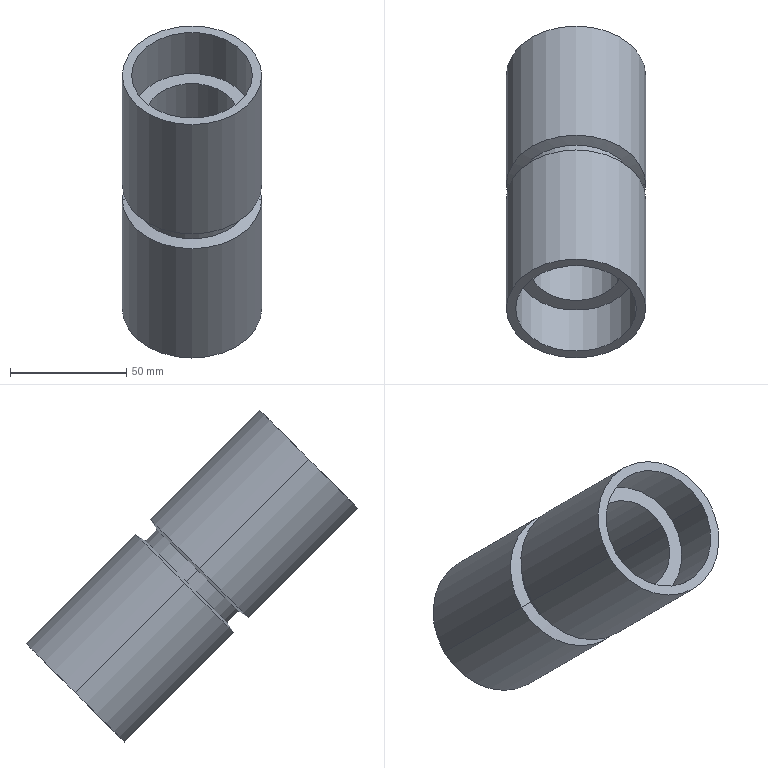Component | SolidWorks | PassiveRollerAssembly-1_StainlessSteelRoller-2 | 1 solid | 20 faces | box 60 x 142.84 x 142.84 mm | volume 167559 mm3 | cylinder 12 | cone 4 | plane 4 | commonest cylinder face diameters 52 x4 60 x4 40 x2 50 x2
build123d program:
from build123d import *


with BuildPart() as part:
    # Sketch1 → Revolve1 (revolve)
    with BuildSketch(Plane.XY, mode=Mode.PRIVATE) as revolve1_sk:
        Polygon((0, 26), (0, 30), (66.5, 30), (67.5, 25), (74.5, 25), (75.5, 30), (142, 30), (142, 26), (111, 26), (111, 20), (25, 20), (25, 26), align=None)
    revolve(revolve1_sk.sketch.rotate(Axis((-104.65, 0, 0), (1, 0, 0)), 90), axis=Axis((-104.65, 0, 0), (1, 0, 0)))


solid = part.part

# Placed as in the assembly
solid = solid.moved(Location((2216.026, 658.479, 246.908), (-45, -12.915, 90)))
STEP:
#1=COLOUR_RGB('',0.7922,0.8196,0.9333);
#2=FILL_AREA_STYLE_COLOUR('',#1);
#3=FILL_AREA_STYLE('',(#2));
#4=SURFACE_STYLE_FILL_AREA(#3);
#5=SURFACE_SIDE_STYLE('',(#4));
#6=SURFACE_STYLE_USAGE(.BOTH.,#5);
#7=PRESENTATION_STYLE_ASSIGNMENT((#6));
#8=CARTESIAN_POINT('',(86.458,29.014,6.631));
#9=VERTEX_POINT('',#8);
#10=CARTESIAN_POINT('',(88.033,29.014,6.631));
#11=VERTEX_POINT('',#10);
#12=CARTESIAN_POINT('',(87.245,29.014,6.631));
#13=DIRECTION('',(0.,-0.7071,0.7071));
#14=DIRECTION('',(1.,0.,0.));
#15=AXIS2_PLACEMENT_3D('',#12,#13,#14);
#16=CIRCLE('',#15,0.7874);
#17=EDGE_CURVE('',#9,#11,#16,.T.);
#18=ORIENTED_EDGE('',*,*,#17,.F.);
#19=CARTESIAN_POINT('',(86.458,26.62,9.025));
#20=VERTEX_POINT('',#19);
#21=CARTESIAN_POINT('',(86.458,23.011,12.634));
#22=DIRECTION('',(0.,-0.7071,0.7071));
#23=VECTOR('',#22,39.37);
#24=LINE('',#21,#23);
#25=EDGE_CURVE('',#9,#20,#24,.T.);
#26=ORIENTED_EDGE('',*,*,#25,.T.);
#27=CARTESIAN_POINT('',(88.033,26.62,9.025));
#28=VERTEX_POINT('',#27);
#29=CARTESIAN_POINT('',(87.245,26.62,9.025));
#30=DIRECTION('',(0.,-0.7071,0.7071));
#31=DIRECTION('',(1.,0.,0.));
#32=AXIS2_PLACEMENT_3D('',#29,#30,#31);
#33=CIRCLE('',#32,0.7874);
#34=EDGE_CURVE('',#20,#28,#33,.T.);
#35=ORIENTED_EDGE('',*,*,#34,.T.);
#36=CARTESIAN_POINT('',(88.033,23.011,12.634));
#37=DIRECTION('',(0.,-0.7071,0.7071));
#38=VECTOR('',#37,39.37);
#39=LINE('',#36,#38);
#40=EDGE_CURVE('',#11,#28,#39,.T.);
#41=ORIENTED_EDGE('',*,*,#40,.F.);
#42=EDGE_LOOP('',(#18,#26,#35,#41));
#43=FACE_OUTER_BOUND('',#42,.T.);
#44=CARTESIAN_POINT('',(87.245,23.011,12.634));
#45=DIRECTION('',(0.,-0.7071,0.7071));
#46=DIRECTION('',(1.,0.,0.));
#47=AXIS2_PLACEMENT_3D('',#44,#45,#46);
#48=CYLINDRICAL_SURFACE('',#47,0.7874);
#49=ADVANCED_FACE('',(#43),#48,.F.);
#50=CARTESIAN_POINT('',(86.222,29.877,5.768));
#51=VERTEX_POINT('',#50);
#52=CARTESIAN_POINT('',(88.269,29.877,5.768));
#53=VERTEX_POINT('',#52);
#54=CARTESIAN_POINT('',(87.245,29.877,5.768));
#55=DIRECTION('',(0.,-0.7071,0.7071));
#56=DIRECTION('',(1.,0.,0.));
#57=AXIS2_PLACEMENT_3D('',#54,#55,#56);
#58=CIRCLE('',#57,1.024);
#59=EDGE_CURVE('',#51,#53,#58,.T.);
#60=ORIENTED_EDGE('',*,*,#59,.F.);
#61=CARTESIAN_POINT('',(86.222,29.014,6.631));
#62=VERTEX_POINT('',#61);
#63=CARTESIAN_POINT('',(86.222,23.011,12.634));
#64=DIRECTION('',(0.,-0.7071,0.7071));
#65=VECTOR('',#64,39.37);
#66=LINE('',#63,#65);
#67=EDGE_CURVE('',#51,#62,#66,.T.);
#68=ORIENTED_EDGE('',*,*,#67,.T.);
#69=CARTESIAN_POINT('',(88.269,29.014,6.631));
#70=VERTEX_POINT('',#69);
#71=CARTESIAN_POINT('',(87.245,29.014,6.631));
#72=DIRECTION('',(0.,-0.7071,0.7071));
#73=DIRECTION('',(1.,0.,0.));
#74=AXIS2_PLACEMENT_3D('',#71,#72,#73);
#75=CIRCLE('',#74,1.024);
#76=EDGE_CURVE('',#62,#70,#75,.T.);
#77=ORIENTED_EDGE('',*,*,#76,.T.);
#78=CARTESIAN_POINT('',(88.269,23.011,12.634));
#79=DIRECTION('',(0.,-0.7071,0.7071));
#80=VECTOR('',#79,39.37);
#81=LINE('',#78,#80);
#82=EDGE_CURVE('',#53,#70,#81,.T.);
#83=ORIENTED_EDGE('',*,*,#82,.F.);
#84=EDGE_LOOP('',(#60,#68,#77,#83));
#85=FACE_OUTER_BOUND('',#84,.T.);
#86=CARTESIAN_POINT('',(87.245,23.011,12.634));
#87=DIRECTION('',(0.,-0.7071,0.7071));
#88=DIRECTION('',(1.,0.,0.));
#89=AXIS2_PLACEMENT_3D('',#86,#87,#88);
#90=CYLINDRICAL_SURFACE('',#89,1.024);
#91=ADVANCED_FACE('',(#85),#90,.F.);
#92=CARTESIAN_POINT('',(88.426,29.877,5.768));
#93=VERTEX_POINT('',#92);
#94=CARTESIAN_POINT('',(86.064,29.877,5.768));
#95=VERTEX_POINT('',#94);
#96=CARTESIAN_POINT('',(87.245,29.877,5.768));
#97=DIRECTION('',(0.,-0.7071,0.7071));
#98=DIRECTION('',(1.,0.,0.));
#99=AXIS2_PLACEMENT_3D('',#96,#97,#98);
#100=CIRCLE('',#99,1.181);
#101=EDGE_CURVE('',#93,#95,#100,.T.);
#102=ORIENTED_EDGE('',*,*,#101,.T.);
#103=CARTESIAN_POINT('',(86.064,28.026,7.619));
#104=VERTEX_POINT('',#103);
#105=CARTESIAN_POINT('',(86.064,23.011,12.634));
#106=DIRECTION('',(0.,-0.7071,0.7071));
#107=VECTOR('',#106,39.37);
#108=LINE('',#105,#107);
#109=EDGE_CURVE('',#95,#104,#108,.T.);
#110=ORIENTED_EDGE('',*,*,#109,.T.);
#111=CARTESIAN_POINT('',(88.426,28.026,7.619));
#112=VERTEX_POINT('',#111);
#113=CARTESIAN_POINT('',(87.245,28.026,7.619));
#114=DIRECTION('',(0.,-0.7071,0.7071));
#115=DIRECTION('',(1.,0.,0.));
#116=AXIS2_PLACEMENT_3D('',#113,#114,#115);
#117=CIRCLE('',#116,1.181);
#118=EDGE_CURVE('',#112,#104,#117,.T.);
#119=ORIENTED_EDGE('',*,*,#118,.F.);
#120=CARTESIAN_POINT('',(88.426,23.011,12.634));
#121=DIRECTION('',(0.,-0.7071,0.7071));
#122=VECTOR('',#121,39.37);
#123=LINE('',#120,#122);
#124=EDGE_CURVE('',#93,#112,#123,.T.);
#125=ORIENTED_EDGE('',*,*,#124,.F.);
#126=EDGE_LOOP('',(#102,#110,#119,#125));
#127=FACE_OUTER_BOUND('',#126,.T.);
#128=CARTESIAN_POINT('',(87.245,23.011,12.634));
#129=DIRECTION('',(0.,-0.7071,0.7071));
#130=DIRECTION('',(1.,0.,0.));
#131=AXIS2_PLACEMENT_3D('',#128,#129,#130);
#132=CYLINDRICAL_SURFACE('',#131,1.181);
#133=ADVANCED_FACE('',(#127),#132,.T.);
#134=CARTESIAN_POINT('',(88.229,27.998,7.647));
#135=VERTEX_POINT('',#134);
#136=CARTESIAN_POINT('',(86.261,27.998,7.647));
#137=VERTEX_POINT('',#136);
#138=CARTESIAN_POINT('',(87.245,27.998,7.647));
#139=DIRECTION('',(0.,-0.7071,0.7071));
#140=DIRECTION('',(1.,0.,0.));
#141=AXIS2_PLACEMENT_3D('',#138,#139,#140);
#142=CIRCLE('',#141,0.9843);
#143=EDGE_CURVE('',#135,#137,#142,.T.);
#144=ORIENTED_EDGE('',*,*,#143,.F.);
#145=CARTESIAN_POINT('',(88.426,28.026,7.619));
#146=DIRECTION('',(0.9806,0.1387,-0.1387));
#147=VECTOR('',#146,39.37);
#148=LINE('',#145,#147);
#149=EDGE_CURVE('',#135,#112,#148,.T.);
#150=ORIENTED_EDGE('',*,*,#149,.T.);
#151=ORIENTED_EDGE('',*,*,#118,.T.);
#152=CARTESIAN_POINT('',(86.064,28.026,7.619));
#153=DIRECTION('',(-0.9806,0.1387,-0.1387));
#154=VECTOR('',#153,39.37);
#155=LINE('',#152,#154);
#156=EDGE_CURVE('',#137,#104,#155,.T.);
#157=ORIENTED_EDGE('',*,*,#156,.F.);
#158=EDGE_LOOP('',(#144,#150,#151,#157));
#159=FACE_OUTER_BOUND('',#158,.T.);
#160=CARTESIAN_POINT('',(87.245,28.026,7.619));
#161=DIRECTION('',(-0.,0.7071,-0.7071));
#162=DIRECTION('',(-1.,0.,0.));
#163=AXIS2_PLACEMENT_3D('',#160,#161,#162);
#164=CONICAL_SURFACE('',#163,1.181,1.373);
#165=ADVANCED_FACE('',(#159),#164,.T.);
#166=ORIENTED_EDGE('',*,*,#143,.T.);
#167=CARTESIAN_POINT('',(86.261,27.803,7.842));
#168=VERTEX_POINT('',#167);
#169=CARTESIAN_POINT('',(86.261,23.011,12.634));
#170=DIRECTION('',(0.,-0.7071,0.7071));
#171=VECTOR('',#170,39.37);
#172=LINE('',#169,#171);
#173=EDGE_CURVE('',#137,#168,#172,.T.);
#174=ORIENTED_EDGE('',*,*,#173,.T.);
#175=CARTESIAN_POINT('',(88.229,27.803,7.842));
#176=VERTEX_POINT('',#175);
#177=CARTESIAN_POINT('',(87.245,27.803,7.842));
#178=DIRECTION('',(0.,-0.7071,0.7071));
#179=DIRECTION('',(1.,0.,0.));
#180=AXIS2_PLACEMENT_3D('',#177,#178,#179);
#181=CIRCLE('',#180,0.9843);
#182=EDGE_CURVE('',#176,#168,#181,.T.);
#183=ORIENTED_EDGE('',*,*,#182,.F.);
#184=CARTESIAN_POINT('',(88.229,23.011,12.634));
#185=DIRECTION('',(0.,-0.7071,0.7071));
#186=VECTOR('',#185,39.37);
#187=LINE('',#184,#186);
#188=EDGE_CURVE('',#135,#176,#187,.T.);
#189=ORIENTED_EDGE('',*,*,#188,.F.);
#190=EDGE_LOOP('',(#166,#174,#183,#189));
#191=FACE_OUTER_BOUND('',#190,.T.);
#192=CARTESIAN_POINT('',(87.245,23.011,12.634));
#193=DIRECTION('',(0.,-0.7071,0.7071));
#194=DIRECTION('',(1.,0.,0.));
#195=AXIS2_PLACEMENT_3D('',#192,#193,#194);
#196=CYLINDRICAL_SURFACE('',#195,0.9843);
#197=ADVANCED_FACE('',(#191),#196,.T.);
#198=ORIENTED_EDGE('',*,*,#182,.T.);
#199=CARTESIAN_POINT('',(86.064,27.776,7.87));
#200=VERTEX_POINT('',#199);
#201=CARTESIAN_POINT('',(86.261,27.803,7.842));
#202=DIRECTION('',(-0.9806,-0.1387,0.1387));
#203=VECTOR('',#202,39.37);
#204=LINE('',#201,#203);
#205=EDGE_CURVE('',#168,#200,#204,.T.);
#206=ORIENTED_EDGE('',*,*,#205,.T.);
#207=CARTESIAN_POINT('',(88.426,27.776,7.87));
#208=VERTEX_POINT('',#207);
#209=CARTESIAN_POINT('',(87.245,27.776,7.87));
#210=DIRECTION('',(0.,-0.7071,0.7071));
#211=DIRECTION('',(1.,0.,0.));
#212=AXIS2_PLACEMENT_3D('',#209,#210,#211);
#213=CIRCLE('',#212,1.181);
#214=EDGE_CURVE('',#208,#200,#213,.T.);
#215=ORIENTED_EDGE('',*,*,#214,.F.);
#216=CARTESIAN_POINT('',(88.229,27.803,7.842));
#217=DIRECTION('',(0.9806,-0.1387,0.1387));
#218=VECTOR('',#217,39.37);
#219=LINE('',#216,#218);
#220=EDGE_CURVE('',#176,#208,#219,.T.);
#221=ORIENTED_EDGE('',*,*,#220,.F.);
#222=EDGE_LOOP('',(#198,#206,#215,#221));
#223=FACE_OUTER_BOUND('',#222,.T.);
#224=CARTESIAN_POINT('',(87.245,27.803,7.842));
#225=DIRECTION('',(0.,-0.7071,0.7071));
#226=DIRECTION('',(1.,0.,0.));
#227=AXIS2_PLACEMENT_3D('',#224,#225,#226);
#228=CONICAL_SURFACE('',#227,0.9843,1.373);
#229=ADVANCED_FACE('',(#223),#228,.T.);
#230=ORIENTED_EDGE('',*,*,#214,.T.);
#231=CARTESIAN_POINT('',(86.064,25.924,9.721));
#232=VERTEX_POINT('',#231);
#233=CARTESIAN_POINT('',(86.064,23.011,12.634));
#234=DIRECTION('',(0.,-0.7071,0.7071));
#235=VECTOR('',#234,39.37);
#236=LINE('',#233,#235);
#237=EDGE_CURVE('',#200,#232,#236,.T.);
#238=ORIENTED_EDGE('',*,*,#237,.T.);
#239=CARTESIAN_POINT('',(88.426,25.924,9.721));
#240=VERTEX_POINT('',#239);
#241=CARTESIAN_POINT('',(87.245,25.924,9.721));
#242=DIRECTION('',(0.,-0.7071,0.7071));
#243=DIRECTION('',(1.,0.,0.));
#244=AXIS2_PLACEMENT_3D('',#241,#242,#243);
#245=CIRCLE('',#244,1.181);
#246=EDGE_CURVE('',#240,#232,#245,.T.);
#247=ORIENTED_EDGE('',*,*,#246,.F.);
#248=CARTESIAN_POINT('',(88.426,23.011,12.634));
#249=DIRECTION('',(0.,-0.7071,0.7071));
#250=VECTOR('',#249,39.37);
#251=LINE('',#248,#250);
#252=EDGE_CURVE('',#208,#240,#251,.T.);
#253=ORIENTED_EDGE('',*,*,#252,.F.);
#254=EDGE_LOOP('',(#230,#238,#247,#253));
#255=FACE_OUTER_BOUND('',#254,.T.);
#256=CARTESIAN_POINT('',(87.245,23.011,12.634));
#257=DIRECTION('',(0.,-0.7071,0.7071));
#258=DIRECTION('',(1.,0.,0.));
#259=AXIS2_PLACEMENT_3D('',#256,#257,#258);
#260=CYLINDRICAL_SURFACE('',#259,1.181);
#261=ADVANCED_FACE('',(#255),#260,.T.);
#262=CARTESIAN_POINT('',(86.222,26.62,9.025));
#263=VERTEX_POINT('',#262);
#264=CARTESIAN_POINT('',(88.269,26.62,9.025));
#265=VERTEX_POINT('',#264);
#266=CARTESIAN_POINT('',(87.245,26.62,9.025));
#267=DIRECTION('',(0.,-0.7071,0.7071));
#268=DIRECTION('',(1.,0.,0.));
#269=AXIS2_PLACEMENT_3D('',#266,#267,#268);
#270=CIRCLE('',#269,1.024);
#271=EDGE_CURVE('',#263,#265,#270,.T.);
#272=ORIENTED_EDGE('',*,*,#271,.F.);
#273=CARTESIAN_POINT('',(86.222,25.924,9.721));
#274=VERTEX_POINT('',#273);
#275=CARTESIAN_POINT('',(86.222,23.011,12.634));
#276=DIRECTION('',(0.,-0.7071,0.7071));
#277=VECTOR('',#276,39.37);
#278=LINE('',#275,#277);
#279=EDGE_CURVE('',#263,#274,#278,.T.);
#280=ORIENTED_EDGE('',*,*,#279,.T.);
#281=CARTESIAN_POINT('',(88.269,25.924,9.721));
#282=VERTEX_POINT('',#281);
#283=CARTESIAN_POINT('',(87.245,25.924,9.721));
#284=DIRECTION('',(0.,-0.7071,0.7071));
#285=DIRECTION('',(1.,0.,0.));
#286=AXIS2_PLACEMENT_3D('',#283,#284,#285);
#287=CIRCLE('',#286,1.024);
#288=EDGE_CURVE('',#274,#282,#287,.T.);
#289=ORIENTED_EDGE('',*,*,#288,.T.);
#290=CARTESIAN_POINT('',(88.269,23.011,12.634));
#291=DIRECTION('',(0.,-0.7071,0.7071));
#292=VECTOR('',#291,39.37);
#293=LINE('',#290,#292);
#294=EDGE_CURVE('',#265,#282,#293,.T.);
#295=ORIENTED_EDGE('',*,*,#294,.F.);
#296=EDGE_LOOP('',(#272,#280,#289,#295));
#297=FACE_OUTER_BOUND('',#296,.T.);
#298=CARTESIAN_POINT('',(87.245,23.011,12.634));
#299=DIRECTION('',(0.,-0.7071,0.7071));
#300=DIRECTION('',(1.,0.,0.));
#301=AXIS2_PLACEMENT_3D('',#298,#299,#300);
#302=CYLINDRICAL_SURFACE('',#301,1.024);
#303=ADVANCED_FACE('',(#297),#302,.F.);
#304=ORIENTED_EDGE('',*,*,#279,.F.);
#305=CARTESIAN_POINT('',(87.245,26.62,9.025));
#306=DIRECTION('',(0.,-0.7071,0.7071));
#307=DIRECTION('',(1.,0.,0.));
#308=AXIS2_PLACEMENT_3D('',#305,#306,#307);
#309=CIRCLE('',#308,1.024);
#310=EDGE_CURVE('',#265,#263,#309,.T.);
#311=ORIENTED_EDGE('',*,*,#310,.F.);
#312=ORIENTED_EDGE('',*,*,#294,.T.);
#313=CARTESIAN_POINT('',(87.245,25.924,9.721));
#314=DIRECTION('',(0.,-0.7071,0.7071));
#315=DIRECTION('',(1.,0.,0.));
#316=AXIS2_PLACEMENT_3D('',#313,#314,#315);
#317=CIRCLE('',#316,1.024);
#318=EDGE_CURVE('',#282,#274,#317,.T.);
#319=ORIENTED_EDGE('',*,*,#318,.T.);
#320=EDGE_LOOP('',(#304,#311,#312,#319));
#321=FACE_OUTER_BOUND('',#320,.T.);
#322=CARTESIAN_POINT('',(87.245,23.011,12.634));
#323=DIRECTION('',(0.,-0.7071,0.7071));
#324=DIRECTION('',(1.,0.,0.));
#325=AXIS2_PLACEMENT_3D('',#322,#323,#324);
#326=CYLINDRICAL_SURFACE('',#325,1.024);
#327=ADVANCED_FACE('',(#321),#326,.F.);
#328=ORIENTED_EDGE('',*,*,#318,.F.);
#329=ORIENTED_EDGE('',*,*,#288,.F.);
#330=EDGE_LOOP('',(#328,#329));
#331=FACE_BOUND('',#330,.T.);
#332=ORIENTED_EDGE('',*,*,#246,.T.);
#333=CARTESIAN_POINT('',(87.245,25.924,9.721));
#334=DIRECTION('',(0.,-0.7071,0.7071));
#335=DIRECTION('',(1.,0.,0.));
#336=AXIS2_PLACEMENT_3D('',#333,#334,#335);
#337=CIRCLE('',#336,1.181);
#338=EDGE_CURVE('',#232,#240,#337,.T.);
#339=ORIENTED_EDGE('',*,*,#338,.T.);
#340=EDGE_LOOP('',(#332,#339));
#341=FACE_OUTER_BOUND('',#340,.T.);
#342=CARTESIAN_POINT('',(87.245,26.648,10.445));
#343=DIRECTION('',(-0.,0.7071,-0.7071));
#344=DIRECTION('',(-1.,0.,0.));
#345=AXIS2_PLACEMENT_3D('',#342,#343,#344);
#346=PLANE('',#345);
#347=ADVANCED_FACE('',(#331,#341),#346,.F.);
#348=ORIENTED_EDGE('',*,*,#237,.F.);
#349=CARTESIAN_POINT('',(87.245,27.776,7.87));
#350=DIRECTION('',(0.,-0.7071,0.7071));
#351=DIRECTION('',(1.,0.,0.));
#352=AXIS2_PLACEMENT_3D('',#349,#350,#351);
#353=CIRCLE('',#352,1.181);
#354=EDGE_CURVE('',#200,#208,#353,.T.);
#355=ORIENTED_EDGE('',*,*,#354,.T.);
#356=ORIENTED_EDGE('',*,*,#252,.T.);
#357=ORIENTED_EDGE('',*,*,#338,.F.);
#358=EDGE_LOOP('',(#348,#355,#356,#357));
#359=FACE_OUTER_BOUND('',#358,.T.);
#360=CARTESIAN_POINT('',(87.245,23.011,12.634));
#361=DIRECTION('',(0.,-0.7071,0.7071));
#362=DIRECTION('',(1.,0.,0.));
#363=AXIS2_PLACEMENT_3D('',#360,#361,#362);
#364=CYLINDRICAL_SURFACE('',#363,1.181);
#365=ADVANCED_FACE('',(#359),#364,.T.);
#366=ORIENTED_EDGE('',*,*,#205,.F.);
#367=CARTESIAN_POINT('',(87.245,27.803,7.842));
#368=DIRECTION('',(0.,-0.7071,0.7071));
#369=DIRECTION('',(1.,0.,0.));
#370=AXIS2_PLACEMENT_3D('',#367,#368,#369);
#371=CIRCLE('',#370,0.9843);
#372=EDGE_CURVE('',#168,#176,#371,.T.);
#373=ORIENTED_EDGE('',*,*,#372,.T.);
#374=ORIENTED_EDGE('',*,*,#220,.T.);
#375=ORIENTED_EDGE('',*,*,#354,.F.);
#376=EDGE_LOOP('',(#366,#373,#374,#375));
#377=FACE_OUTER_BOUND('',#376,.T.);
#378=CARTESIAN_POINT('',(87.245,27.803,7.842));
#379=DIRECTION('',(0.,-0.7071,0.7071));
#380=DIRECTION('',(1.,0.,0.));
#381=AXIS2_PLACEMENT_3D('',#378,#379,#380);
#382=CONICAL_SURFACE('',#381,0.9843,1.373);
#383=ADVANCED_FACE('',(#377),#382,.T.);
#384=ORIENTED_EDGE('',*,*,#173,.F.);
#385=CARTESIAN_POINT('',(87.245,27.998,7.647));
#386=DIRECTION('',(0.,-0.7071,0.7071));
#387=DIRECTION('',(1.,0.,0.));
#388=AXIS2_PLACEMENT_3D('',#385,#386,#387);
#389=CIRCLE('',#388,0.9843);
#390=EDGE_CURVE('',#137,#135,#389,.T.);
#391=ORIENTED_EDGE('',*,*,#390,.T.);
#392=ORIENTED_EDGE('',*,*,#188,.T.);
#393=ORIENTED_EDGE('',*,*,#372,.F.);
#394=EDGE_LOOP('',(#384,#391,#392,#393));
#395=FACE_OUTER_BOUND('',#394,.T.);
#396=CARTESIAN_POINT('',(87.245,23.011,12.634));
#397=DIRECTION('',(0.,-0.7071,0.7071));
#398=DIRECTION('',(1.,0.,0.));
#399=AXIS2_PLACEMENT_3D('',#396,#397,#398);
#400=CYLINDRICAL_SURFACE('',#399,0.9843);
#401=ADVANCED_FACE('',(#395),#400,.T.);
#402=ORIENTED_EDGE('',*,*,#149,.F.);
#403=ORIENTED_EDGE('',*,*,#390,.F.);
#404=ORIENTED_EDGE('',*,*,#156,.T.);
#405=CARTESIAN_POINT('',(87.245,28.026,7.619));
#406=DIRECTION('',(0.,-0.7071,0.7071));
#407=DIRECTION('',(1.,0.,0.));
#408=AXIS2_PLACEMENT_3D('',#405,#406,#407);
#409=CIRCLE('',#408,1.181);
#410=EDGE_CURVE('',#104,#112,#409,.T.);
#411=ORIENTED_EDGE('',*,*,#410,.T.);
#412=EDGE_LOOP('',(#402,#403,#404,#411));
#413=FACE_OUTER_BOUND('',#412,.T.);
#414=CARTESIAN_POINT('',(87.245,28.026,7.619));
#415=DIRECTION('',(-0.,0.7071,-0.7071));
#416=DIRECTION('',(-1.,0.,0.));
#417=AXIS2_PLACEMENT_3D('',#414,#415,#416);
#418=CONICAL_SURFACE('',#417,1.181,1.373);
#419=ADVANCED_FACE('',(#413),#418,.T.);
#420=ORIENTED_EDGE('',*,*,#109,.F.);
#421=CARTESIAN_POINT('',(87.245,29.877,5.768));
#422=DIRECTION('',(0.,-0.7071,0.7071));
#423=DIRECTION('',(1.,0.,0.));
#424=AXIS2_PLACEMENT_3D('',#421,#422,#423);
#425=CIRCLE('',#424,1.181);
#426=EDGE_CURVE('',#95,#93,#425,.T.);
#427=ORIENTED_EDGE('',*,*,#426,.T.);
#428=ORIENTED_EDGE('',*,*,#124,.T.);
#429=ORIENTED_EDGE('',*,*,#410,.F.);
#430=EDGE_LOOP('',(#420,#427,#428,#429));
#431=FACE_OUTER_BOUND('',#430,.T.);
#432=CARTESIAN_POINT('',(87.245,23.011,12.634));
#433=DIRECTION('',(0.,-0.7071,0.7071));
#434=DIRECTION('',(1.,0.,0.));
#435=AXIS2_PLACEMENT_3D('',#432,#433,#434);
#436=CYLINDRICAL_SURFACE('',#435,1.181);
#437=ADVANCED_FACE('',(#431),#436,.T.);
#438=ORIENTED_EDGE('',*,*,#101,.F.);
#439=ORIENTED_EDGE('',*,*,#426,.F.);
#440=EDGE_LOOP('',(#438,#439));
#441=FACE_OUTER_BOUND('',#440,.T.);
#442=CARTESIAN_POINT('',(87.245,29.877,5.768));
#443=DIRECTION('',(0.,-0.7071,0.7071));
#444=DIRECTION('',(1.,0.,0.));
#445=AXIS2_PLACEMENT_3D('',#442,#443,#444);
#446=CIRCLE('',#445,1.024);
#447=EDGE_CURVE('',#53,#51,#446,.T.);
#448=ORIENTED_EDGE('',*,*,#447,.T.);
#449=ORIENTED_EDGE('',*,*,#59,.T.);
#450=EDGE_LOOP('',(#448,#449));
#451=FACE_BOUND('',#450,.T.);
#452=CARTESIAN_POINT('',(87.245,30.713,6.603));
#453=DIRECTION('',(0.,-0.7071,0.7071));
#454=DIRECTION('',(1.,-0.,-0.));
#455=AXIS2_PLACEMENT_3D('',#452,#453,#454);
#456=PLANE('',#455);
#457=ADVANCED_FACE('',(#441,#451),#456,.F.);
#458=ORIENTED_EDGE('',*,*,#67,.F.);
#459=ORIENTED_EDGE('',*,*,#447,.F.);
#460=ORIENTED_EDGE('',*,*,#82,.T.);
#461=CARTESIAN_POINT('',(87.245,29.014,6.631));
#462=DIRECTION('',(0.,-0.7071,0.7071));
#463=DIRECTION('',(1.,0.,0.));
#464=AXIS2_PLACEMENT_3D('',#461,#462,#463);
#465=CIRCLE('',#464,1.024);
#466=EDGE_CURVE('',#70,#62,#465,.T.);
#467=ORIENTED_EDGE('',*,*,#466,.T.);
#468=EDGE_LOOP('',(#458,#459,#460,#467));
#469=FACE_OUTER_BOUND('',#468,.T.);
#470=CARTESIAN_POINT('',(87.245,23.011,12.634));
#471=DIRECTION('',(0.,-0.7071,0.7071));
#472=DIRECTION('',(1.,0.,0.));
#473=AXIS2_PLACEMENT_3D('',#470,#471,#472);
#474=CYLINDRICAL_SURFACE('',#473,1.024);
#475=ADVANCED_FACE('',(#469),#474,.F.);
#476=ORIENTED_EDGE('',*,*,#466,.F.);
#477=ORIENTED_EDGE('',*,*,#76,.F.);
#478=EDGE_LOOP('',(#476,#477));
#479=FACE_OUTER_BOUND('',#478,.T.);
#480=CARTESIAN_POINT('',(87.245,29.014,6.631));
#481=DIRECTION('',(0.,-0.7071,0.7071));
#482=DIRECTION('',(1.,0.,0.));
#483=AXIS2_PLACEMENT_3D('',#480,#481,#482);
#484=CIRCLE('',#483,0.7874);
#485=EDGE_CURVE('',#11,#9,#484,.T.);
#486=ORIENTED_EDGE('',*,*,#485,.T.);
#487=ORIENTED_EDGE('',*,*,#17,.T.);
#488=EDGE_LOOP('',(#486,#487));
#489=FACE_BOUND('',#488,.T.);
#490=CARTESIAN_POINT('',(87.245,29.738,7.354));
#491=DIRECTION('',(0.,-0.7071,0.7071));
#492=DIRECTION('',(1.,-0.,-0.));
#493=AXIS2_PLACEMENT_3D('',#490,#491,#492);
#494=PLANE('',#493);
#495=ADVANCED_FACE('',(#479,#489),#494,.F.);
#496=ORIENTED_EDGE('',*,*,#25,.F.);
#497=ORIENTED_EDGE('',*,*,#485,.F.);
#498=ORIENTED_EDGE('',*,*,#40,.T.);
#499=CARTESIAN_POINT('',(87.245,26.62,9.025));
#500=DIRECTION('',(0.,-0.7071,0.7071));
#501=DIRECTION('',(1.,0.,0.));
#502=AXIS2_PLACEMENT_3D('',#499,#500,#501);
#503=CIRCLE('',#502,0.7874);
#504=EDGE_CURVE('',#28,#20,#503,.T.);
#505=ORIENTED_EDGE('',*,*,#504,.T.);
#506=EDGE_LOOP('',(#496,#497,#498,#505));
#507=FACE_OUTER_BOUND('',#506,.T.);
#508=CARTESIAN_POINT('',(87.245,23.011,12.634));
#509=DIRECTION('',(0.,-0.7071,0.7071));
#510=DIRECTION('',(1.,0.,0.));
#511=AXIS2_PLACEMENT_3D('',#508,#509,#510);
#512=CYLINDRICAL_SURFACE('',#511,0.7874);
#513=ADVANCED_FACE('',(#507),#512,.F.);
#514=ORIENTED_EDGE('',*,*,#504,.F.);
#515=ORIENTED_EDGE('',*,*,#34,.F.);
#516=EDGE_LOOP('',(#514,#515));
#517=FACE_BOUND('',#516,.T.);
#518=ORIENTED_EDGE('',*,*,#310,.T.);
#519=ORIENTED_EDGE('',*,*,#271,.T.);
#520=EDGE_LOOP('',(#518,#519));
#521=FACE_OUTER_BOUND('',#520,.T.);
#522=CARTESIAN_POINT('',(87.245,27.177,9.582));
#523=DIRECTION('',(-0.,0.7071,-0.7071));
#524=DIRECTION('',(-1.,0.,0.));
#525=AXIS2_PLACEMENT_3D('',#522,#523,#524);
#526=PLANE('',#525);
#527=ADVANCED_FACE('',(#517,#521),#526,.F.);
#528=CLOSED_SHELL('',(#49,#91,#133,#165,#197,#229,#261,#303,#327,#347,#365,#383,#401,#419,#437,#457,#475,#495,#513,#527));
#529=MANIFOLD_SOLID_BREP('',#528);
#530=STYLED_ITEM('',(#7),#529);
#531=PRESENTATION_LAYER_ASSIGNMENT('','',(#530));
#532=(LENGTH_UNIT()NAMED_UNIT(*)SI_UNIT($,.METRE.));
#533=LENGTH_MEASURE_WITH_UNIT(LENGTH_MEASURE(0.0254),#532);
#534=DIMENSIONAL_EXPONENTS(1.,0.,0.,0.,0.,0.,0.);
#535=(CONVERSION_BASED_UNIT('',#533)LENGTH_UNIT()NAMED_UNIT(#534));
#536=UNCERTAINTY_MEASURE_WITH_UNIT(LENGTH_MEASURE(0.00001),#535,'','');
#537=(NAMED_UNIT(*)PLANE_ANGLE_UNIT()SI_UNIT($,.RADIAN.));
#538=(NAMED_UNIT(*)SI_UNIT($,.STERADIAN.)SOLID_ANGLE_UNIT());
#539=(GEOMETRIC_REPRESENTATION_CONTEXT(3)GLOBAL_UNCERTAINTY_ASSIGNED_CONTEXT((#536))GLOBAL_UNIT_ASSIGNED_CONTEXT((#535,#537,#538))REPRESENTATION_CONTEXT('',''));
#540=MECHANICAL_DESIGN_GEOMETRIC_PRESENTATION_REPRESENTATION('',(#530),#539);
#541=CARTESIAN_POINT('',(0.,0.,0.));
#542=DIRECTION('',(0.,0.,1.));
#543=DIRECTION('',(1.,0.,0.));
#544=AXIS2_PLACEMENT_3D('',#541,#542,#543);
#545=(LENGTH_UNIT()NAMED_UNIT(*)SI_UNIT($,.METRE.));
#546=LENGTH_MEASURE_WITH_UNIT(LENGTH_MEASURE(0.0254),#545);
#547=DIMENSIONAL_EXPONENTS(1.,0.,0.,0.,0.,0.,0.);
#548=(CONVERSION_BASED_UNIT('',#546)LENGTH_UNIT()NAMED_UNIT(#547));
#549=UNCERTAINTY_MEASURE_WITH_UNIT(LENGTH_MEASURE(0.00001),#548,'','');
#550=(NAMED_UNIT(*)PLANE_ANGLE_UNIT()SI_UNIT($,.RADIAN.));
#551=(NAMED_UNIT(*)SI_UNIT($,.STERADIAN.)SOLID_ANGLE_UNIT());
#552=(GEOMETRIC_REPRESENTATION_CONTEXT(3)GLOBAL_UNCERTAINTY_ASSIGNED_CONTEXT((#549))GLOBAL_UNIT_ASSIGNED_CONTEXT((#548,#550,#551))REPRESENTATION_CONTEXT('',''));
#553=ADVANCED_BREP_SHAPE_REPRESENTATION('',(#529,#544),#552);